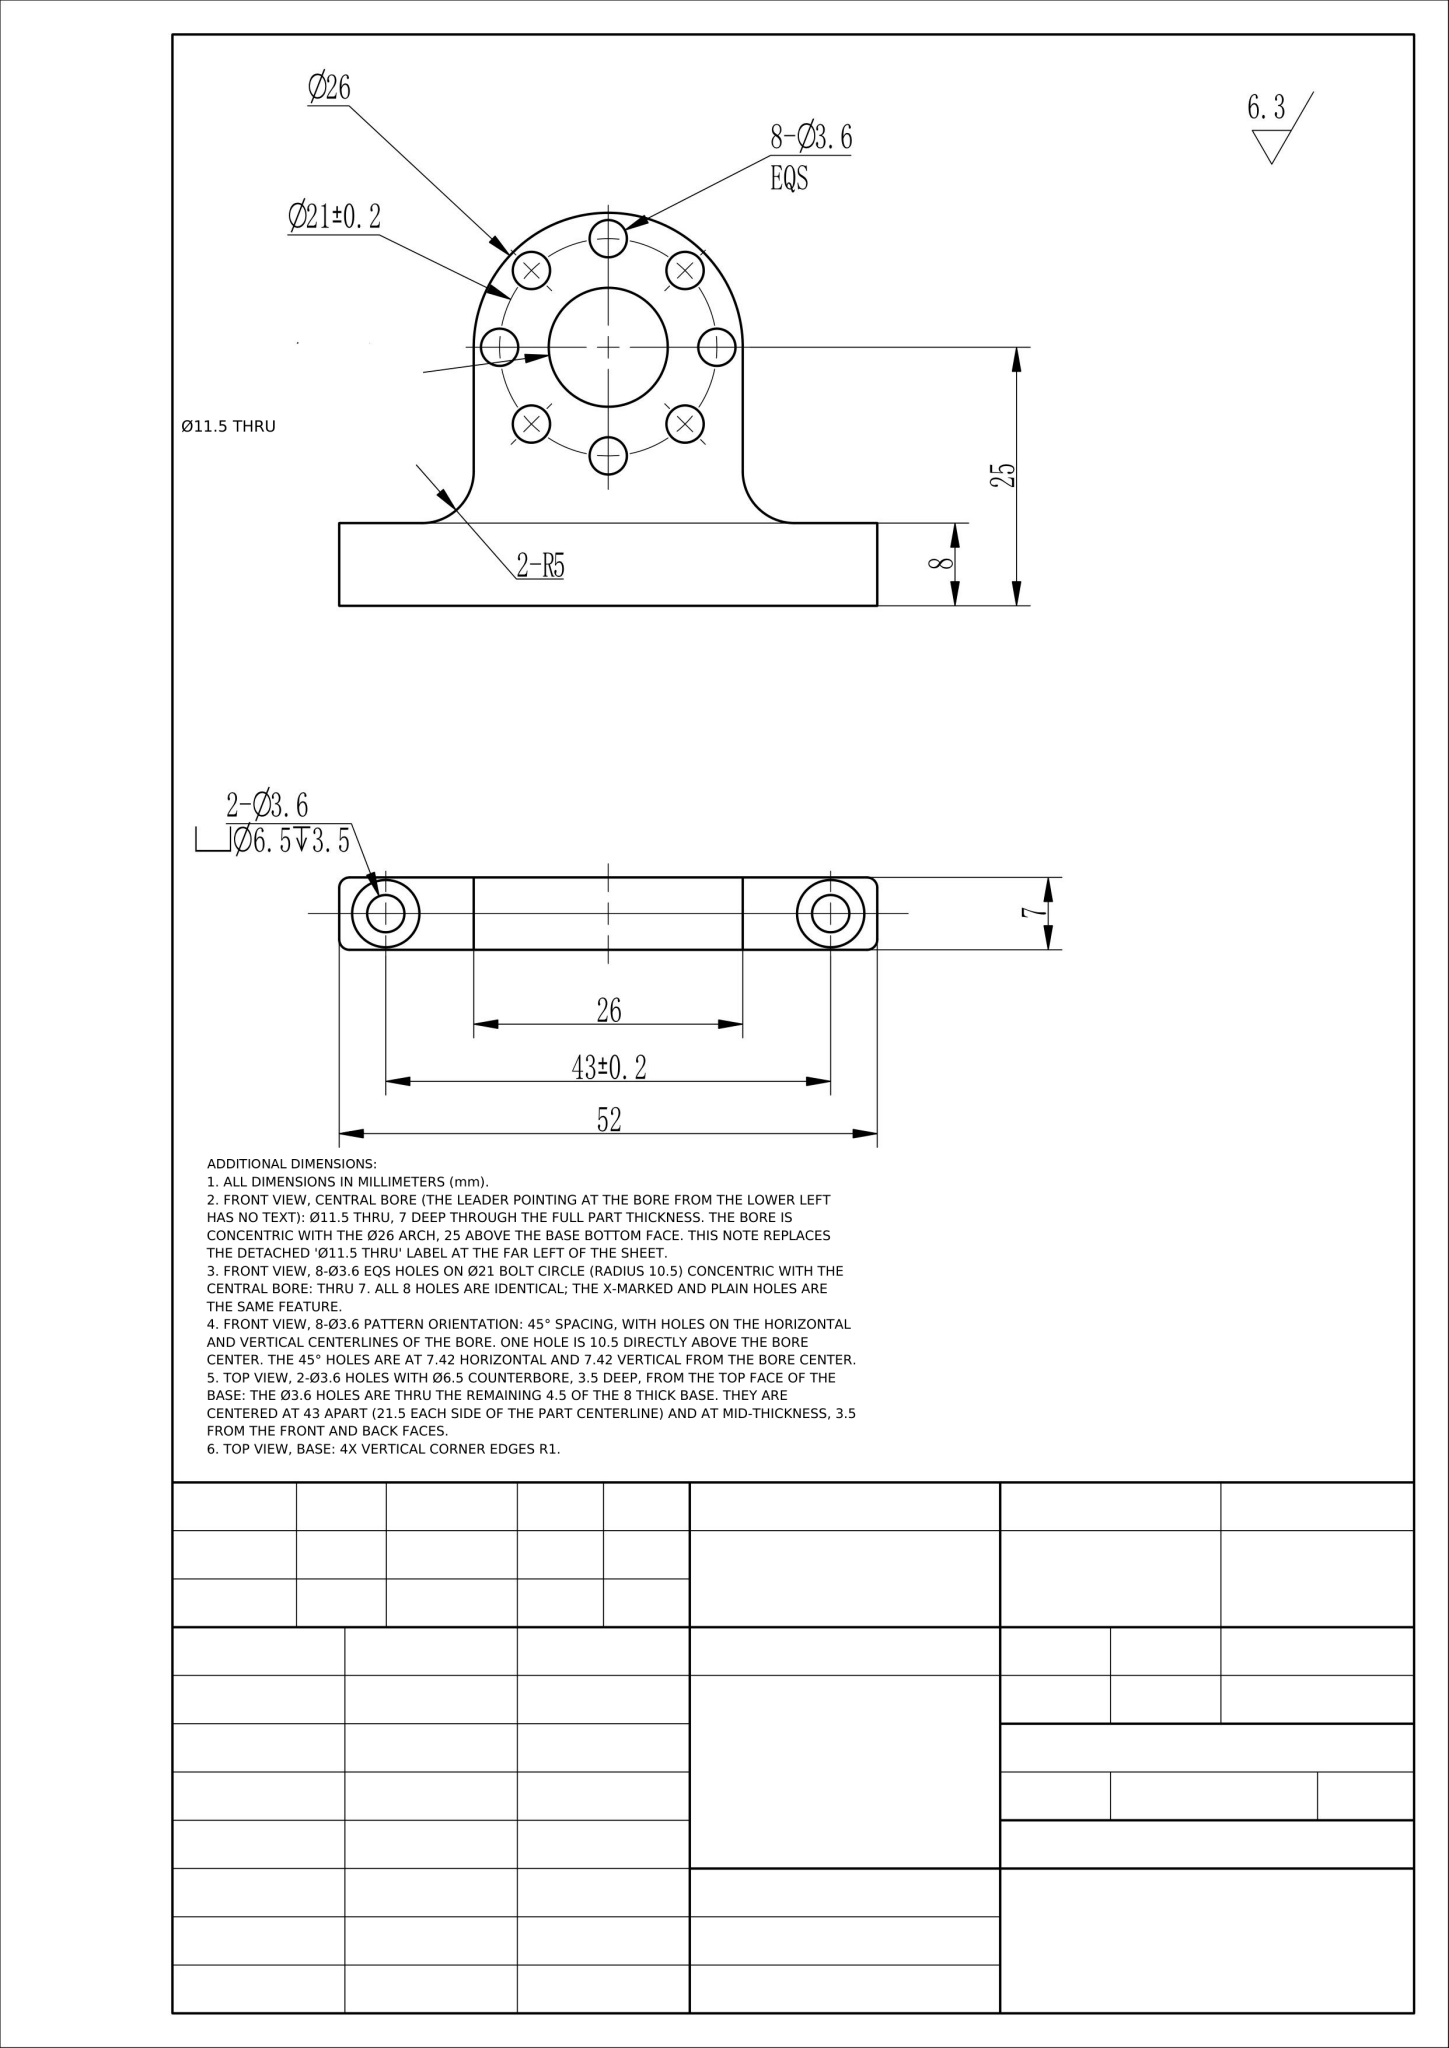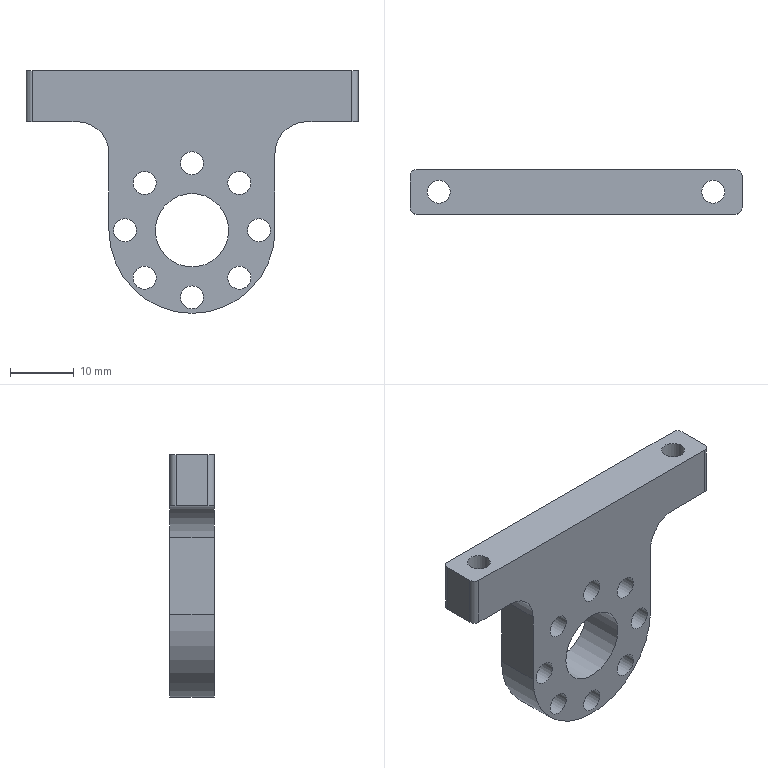Part | NX | mm | 1 solid | 31 faces | box 52 x 7 x 38 mm | volume 6312 mm3 | cylinder 20 | plane 11 | commonest cylinder face diameters 3.6 x10 2 x4 10 x2 6.5 x2 26 x1 11.5 x1
STEP:
#1=CARTESIAN_POINT('',(0.,0.,0.));
#2=DIRECTION('',(0.,0.,1.));
#3=DIRECTION('',(1.,0.,0.));
#4=AXIS2_PLACEMENT_3D('',#1,#2,#3);
#5=(LENGTH_UNIT()NAMED_UNIT(*)SI_UNIT(.MILLI.,.METRE.));
#6=UNCERTAINTY_MEASURE_WITH_UNIT(LENGTH_MEASURE(0.00002),#5,'','');
#7=(NAMED_UNIT(*)PLANE_ANGLE_UNIT()SI_UNIT($,.RADIAN.));
#8=PLANE_ANGLE_MEASURE_WITH_UNIT(PLANE_ANGLE_MEASURE(0.01745),#7);
#9=DIMENSIONAL_EXPONENTS(0.,0.,0.,0.,0.,0.,0.);
#10=(CONVERSION_BASED_UNIT('',#8)NAMED_UNIT(#9)PLANE_ANGLE_UNIT());
#11=(NAMED_UNIT(*)SI_UNIT($,.STERADIAN.)SOLID_ANGLE_UNIT());
#12=(GEOMETRIC_REPRESENTATION_CONTEXT(3)GLOBAL_UNCERTAINTY_ASSIGNED_CONTEXT((#6))GLOBAL_UNIT_ASSIGNED_CONTEXT((#5,#10,#11))REPRESENTATION_CONTEXT('',''));
#13=SHAPE_REPRESENTATION('',(#4),#12);
#14=CARTESIAN_POINT('',(-13.,-7.,-0.));
#15=VERTEX_POINT('',#14);
#16=CARTESIAN_POINT('',(13.,-7.,-0.));
#17=VERTEX_POINT('',#16);
#18=CARTESIAN_POINT('',(0.,-7.,0.));
#19=DIRECTION('',(0.,-1.,0.));
#20=DIRECTION('',(1.,0.,-0.));
#21=AXIS2_PLACEMENT_3D('',#18,#19,#20);
#22=CIRCLE('',#21,13.);
#23=EDGE_CURVE('',#15,#17,#22,.T.);
#24=ORIENTED_EDGE('',*,*,#23,.F.);
#25=CARTESIAN_POINT('',(-13.,0.,-0.));
#26=VERTEX_POINT('',#25);
#27=CARTESIAN_POINT('',(-13.,-7.,0.));
#28=DIRECTION('',(0.,1.,0.));
#29=VECTOR('',#28,1.);
#30=LINE('',#27,#29);
#31=EDGE_CURVE('',#15,#26,#30,.T.);
#32=ORIENTED_EDGE('',*,*,#31,.T.);
#33=CARTESIAN_POINT('',(13.,0.,0.));
#34=VERTEX_POINT('',#33);
#35=CARTESIAN_POINT('',(0.,0.,0.));
#36=DIRECTION('',(0.,-1.,0.));
#37=DIRECTION('',(1.,0.,-0.));
#38=AXIS2_PLACEMENT_3D('',#35,#36,#37);
#39=CIRCLE('',#38,13.);
#40=EDGE_CURVE('',#26,#34,#39,.T.);
#41=ORIENTED_EDGE('',*,*,#40,.T.);
#42=CARTESIAN_POINT('',(13.,-7.,0.));
#43=DIRECTION('',(0.,1.,0.));
#44=VECTOR('',#43,1.);
#45=LINE('',#42,#44);
#46=EDGE_CURVE('',#17,#34,#45,.T.);
#47=ORIENTED_EDGE('',*,*,#46,.F.);
#48=EDGE_LOOP('',(#24,#32,#41,#47));
#49=FACE_OUTER_BOUND('',#48,.T.);
#50=CARTESIAN_POINT('',(0.,0.,0.));
#51=DIRECTION('',(0.,-1.,0.));
#52=DIRECTION('',(0.,0.,-1.));
#53=AXIS2_PLACEMENT_3D('',#50,#51,#52);
#54=CYLINDRICAL_SURFACE('',#53,13.);
#55=ADVANCED_FACE('',(#49),#54,.T.);
#56=CARTESIAN_POINT('',(5.75,0.,-0.));
#57=VERTEX_POINT('',#56);
#58=CARTESIAN_POINT('',(0.,0.,0.));
#59=DIRECTION('',(0.,-1.,0.));
#60=DIRECTION('',(1.,0.,-0.));
#61=AXIS2_PLACEMENT_3D('',#58,#59,#60);
#62=CIRCLE('',#61,5.75);
#63=EDGE_CURVE('',#57,#57,#62,.T.);
#64=ORIENTED_EDGE('',*,*,#63,.F.);
#65=EDGE_LOOP('',(#64));
#66=FACE_BOUND('',#65,.T.);
#67=CARTESIAN_POINT('',(5.75,-7.,-0.));
#68=VERTEX_POINT('',#67);
#69=CARTESIAN_POINT('',(0.,-7.,0.));
#70=DIRECTION('',(0.,-1.,0.));
#71=DIRECTION('',(1.,0.,-0.));
#72=AXIS2_PLACEMENT_3D('',#69,#70,#71);
#73=CIRCLE('',#72,5.75);
#74=EDGE_CURVE('',#68,#68,#73,.T.);
#75=ORIENTED_EDGE('',*,*,#74,.T.);
#76=EDGE_LOOP('',(#75));
#77=FACE_BOUND('',#76,.T.);
#78=CARTESIAN_POINT('',(0.,0.,0.));
#79=DIRECTION('',(0.,-1.,0.));
#80=DIRECTION('',(0.,0.,-1.));
#81=AXIS2_PLACEMENT_3D('',#78,#79,#80);
#82=CYLINDRICAL_SURFACE('',#81,5.75);
#83=ADVANCED_FACE('',(#66,#77),#82,.F.);
#84=CARTESIAN_POINT('',(7.425,0.,5.625));
#85=VERTEX_POINT('',#84);
#86=CARTESIAN_POINT('',(7.425,0.,7.425));
#87=DIRECTION('',(0.,-1.,0.));
#88=DIRECTION('',(0.,0.,-1.));
#89=AXIS2_PLACEMENT_3D('',#86,#87,#88);
#90=CIRCLE('',#89,1.8);
#91=EDGE_CURVE('',#85,#85,#90,.T.);
#92=ORIENTED_EDGE('',*,*,#91,.T.);
#93=EDGE_LOOP('',(#92));
#94=FACE_BOUND('',#93,.T.);
#95=CARTESIAN_POINT('',(10.5,0.,-1.8));
#96=VERTEX_POINT('',#95);
#97=CARTESIAN_POINT('',(10.5,0.,-0.));
#98=DIRECTION('',(0.,-1.,0.));
#99=DIRECTION('',(0.,0.,-1.));
#100=AXIS2_PLACEMENT_3D('',#97,#98,#99);
#101=CIRCLE('',#100,1.8);
#102=EDGE_CURVE('',#96,#96,#101,.T.);
#103=ORIENTED_EDGE('',*,*,#102,.T.);
#104=EDGE_LOOP('',(#103));
#105=FACE_BOUND('',#104,.T.);
#106=CARTESIAN_POINT('',(7.425,0.,-9.225));
#107=VERTEX_POINT('',#106);
#108=CARTESIAN_POINT('',(7.425,0.,-7.425));
#109=DIRECTION('',(0.,-1.,0.));
#110=DIRECTION('',(0.,0.,-1.));
#111=AXIS2_PLACEMENT_3D('',#108,#109,#110);
#112=CIRCLE('',#111,1.8);
#113=EDGE_CURVE('',#107,#107,#112,.T.);
#114=ORIENTED_EDGE('',*,*,#113,.T.);
#115=EDGE_LOOP('',(#114));
#116=FACE_BOUND('',#115,.T.);
#117=CARTESIAN_POINT('',(0.,0.,-12.3));
#118=VERTEX_POINT('',#117);
#119=CARTESIAN_POINT('',(0.,0.,-10.5));
#120=DIRECTION('',(0.,-1.,0.));
#121=DIRECTION('',(0.,0.,-1.));
#122=AXIS2_PLACEMENT_3D('',#119,#120,#121);
#123=CIRCLE('',#122,1.8);
#124=EDGE_CURVE('',#118,#118,#123,.T.);
#125=ORIENTED_EDGE('',*,*,#124,.T.);
#126=EDGE_LOOP('',(#125));
#127=FACE_BOUND('',#126,.T.);
#128=CARTESIAN_POINT('',(-7.425,0.,-9.225));
#129=VERTEX_POINT('',#128);
#130=CARTESIAN_POINT('',(-7.425,0.,-7.425));
#131=DIRECTION('',(0.,-1.,0.));
#132=DIRECTION('',(0.,0.,-1.));
#133=AXIS2_PLACEMENT_3D('',#130,#131,#132);
#134=CIRCLE('',#133,1.8);
#135=EDGE_CURVE('',#129,#129,#134,.T.);
#136=ORIENTED_EDGE('',*,*,#135,.T.);
#137=EDGE_LOOP('',(#136));
#138=FACE_BOUND('',#137,.T.);
#139=CARTESIAN_POINT('',(-10.5,0.,-1.8));
#140=VERTEX_POINT('',#139);
#141=CARTESIAN_POINT('',(-10.5,0.,0.));
#142=DIRECTION('',(0.,-1.,0.));
#143=DIRECTION('',(0.,0.,-1.));
#144=AXIS2_PLACEMENT_3D('',#141,#142,#143);
#145=CIRCLE('',#144,1.8);
#146=EDGE_CURVE('',#140,#140,#145,.T.);
#147=ORIENTED_EDGE('',*,*,#146,.T.);
#148=EDGE_LOOP('',(#147));
#149=FACE_BOUND('',#148,.T.);
#150=CARTESIAN_POINT('',(-7.425,0.,5.625));
#151=VERTEX_POINT('',#150);
#152=CARTESIAN_POINT('',(-7.425,0.,7.425));
#153=DIRECTION('',(0.,-1.,0.));
#154=DIRECTION('',(0.,0.,-1.));
#155=AXIS2_PLACEMENT_3D('',#152,#153,#154);
#156=CIRCLE('',#155,1.8);
#157=EDGE_CURVE('',#151,#151,#156,.T.);
#158=ORIENTED_EDGE('',*,*,#157,.T.);
#159=EDGE_LOOP('',(#158));
#160=FACE_BOUND('',#159,.T.);
#161=CARTESIAN_POINT('',(0.,0.,8.7));
#162=VERTEX_POINT('',#161);
#163=CARTESIAN_POINT('',(0.,0.,10.5));
#164=DIRECTION('',(0.,-1.,0.));
#165=DIRECTION('',(0.,0.,-1.));
#166=AXIS2_PLACEMENT_3D('',#163,#164,#165);
#167=CIRCLE('',#166,1.8);
#168=EDGE_CURVE('',#162,#162,#167,.T.);
#169=ORIENTED_EDGE('',*,*,#168,.T.);
#170=EDGE_LOOP('',(#169));
#171=FACE_BOUND('',#170,.T.);
#172=CARTESIAN_POINT('',(25.,0.,25.));
#173=VERTEX_POINT('',#172);
#174=CARTESIAN_POINT('',(-25.,0.,25.));
#175=VERTEX_POINT('',#174);
#176=CARTESIAN_POINT('',(26.,0.,25.));
#177=DIRECTION('',(-1.,0.,0.));
#178=VECTOR('',#177,1.);
#179=LINE('',#176,#178);
#180=EDGE_CURVE('',#173,#175,#179,.T.);
#181=ORIENTED_EDGE('',*,*,#180,.F.);
#182=CARTESIAN_POINT('',(25.,0.,17.));
#183=VERTEX_POINT('',#182);
#184=CARTESIAN_POINT('',(25.,0.,0.));
#185=DIRECTION('',(0.,0.,-1.));
#186=VECTOR('',#185,1.);
#187=LINE('',#184,#186);
#188=EDGE_CURVE('',#173,#183,#187,.T.);
#189=ORIENTED_EDGE('',*,*,#188,.T.);
#190=CARTESIAN_POINT('',(18.,0.,17.));
#191=VERTEX_POINT('',#190);
#192=CARTESIAN_POINT('',(13.,0.,17.));
#193=DIRECTION('',(1.,0.,0.));
#194=VECTOR('',#193,1.);
#195=LINE('',#192,#194);
#196=EDGE_CURVE('',#191,#183,#195,.T.);
#197=ORIENTED_EDGE('',*,*,#196,.F.);
#198=CARTESIAN_POINT('',(13.,0.,12.));
#199=VERTEX_POINT('',#198);
#200=CARTESIAN_POINT('',(18.,0.,12.));
#201=DIRECTION('',(0.,-1.,0.));
#202=DIRECTION('',(0.,0.,-1.));
#203=AXIS2_PLACEMENT_3D('',#200,#201,#202);
#204=CIRCLE('',#203,5.);
#205=EDGE_CURVE('',#191,#199,#204,.T.);
#206=ORIENTED_EDGE('',*,*,#205,.T.);
#207=CARTESIAN_POINT('',(13.,0.,0.));
#208=DIRECTION('',(0.,0.,1.));
#209=VECTOR('',#208,1.);
#210=LINE('',#207,#209);
#211=EDGE_CURVE('',#34,#199,#210,.T.);
#212=ORIENTED_EDGE('',*,*,#211,.F.);
#213=ORIENTED_EDGE('',*,*,#40,.F.);
#214=CARTESIAN_POINT('',(-13.,0.,12.));
#215=VERTEX_POINT('',#214);
#216=CARTESIAN_POINT('',(-13.,0.,17.));
#217=DIRECTION('',(0.,0.,-1.));
#218=VECTOR('',#217,1.);
#219=LINE('',#216,#218);
#220=EDGE_CURVE('',#215,#26,#219,.T.);
#221=ORIENTED_EDGE('',*,*,#220,.F.);
#222=CARTESIAN_POINT('',(-18.,0.,17.));
#223=VERTEX_POINT('',#222);
#224=CARTESIAN_POINT('',(-18.,0.,12.));
#225=DIRECTION('',(0.,-1.,0.));
#226=DIRECTION('',(0.,0.,-1.));
#227=AXIS2_PLACEMENT_3D('',#224,#225,#226);
#228=CIRCLE('',#227,5.);
#229=EDGE_CURVE('',#215,#223,#228,.T.);
#230=ORIENTED_EDGE('',*,*,#229,.T.);
#231=CARTESIAN_POINT('',(-25.,0.,17.));
#232=VERTEX_POINT('',#231);
#233=CARTESIAN_POINT('',(-26.,0.,17.));
#234=DIRECTION('',(1.,0.,0.));
#235=VECTOR('',#234,1.);
#236=LINE('',#233,#235);
#237=EDGE_CURVE('',#232,#223,#236,.T.);
#238=ORIENTED_EDGE('',*,*,#237,.F.);
#239=CARTESIAN_POINT('',(-25.,0.,0.));
#240=DIRECTION('',(0.,0.,1.));
#241=VECTOR('',#240,1.);
#242=LINE('',#239,#241);
#243=EDGE_CURVE('',#232,#175,#242,.T.);
#244=ORIENTED_EDGE('',*,*,#243,.T.);
#245=EDGE_LOOP('',(#181,#189,#197,#206,#212,#213,#221,#230,#238,#244));
#246=FACE_BOUND('',#245,.T.);
#247=ORIENTED_EDGE('',*,*,#63,.T.);
#248=EDGE_LOOP('',(#247));
#249=FACE_BOUND('',#248,.T.);
#250=CARTESIAN_POINT('',(0.,0.,0.));
#251=DIRECTION('',(0.,-1.,0.));
#252=DIRECTION('',(0.,0.,-1.));
#253=AXIS2_PLACEMENT_3D('',#250,#251,#252);
#254=PLANE('',#253);
#255=ADVANCED_FACE('',(#94,#105,#116,#127,#138,#149,#160,#171,#246,#249),#254,.F.);
#256=CARTESIAN_POINT('',(7.425,-7.,9.225));
#257=VERTEX_POINT('',#256);
#258=CARTESIAN_POINT('',(7.425,-7.,7.425));
#259=DIRECTION('',(0.,1.,0.));
#260=DIRECTION('',(0.,0.,1.));
#261=AXIS2_PLACEMENT_3D('',#258,#259,#260);
#262=CIRCLE('',#261,1.8);
#263=EDGE_CURVE('',#257,#257,#262,.T.);
#264=ORIENTED_EDGE('',*,*,#263,.T.);
#265=EDGE_LOOP('',(#264));
#266=FACE_BOUND('',#265,.T.);
#267=CARTESIAN_POINT('',(10.5,-7.,1.8));
#268=VERTEX_POINT('',#267);
#269=CARTESIAN_POINT('',(10.5,-7.,-0.));
#270=DIRECTION('',(0.,1.,0.));
#271=DIRECTION('',(0.,0.,1.));
#272=AXIS2_PLACEMENT_3D('',#269,#270,#271);
#273=CIRCLE('',#272,1.8);
#274=EDGE_CURVE('',#268,#268,#273,.T.);
#275=ORIENTED_EDGE('',*,*,#274,.T.);
#276=EDGE_LOOP('',(#275));
#277=FACE_BOUND('',#276,.T.);
#278=CARTESIAN_POINT('',(7.425,-7.,-5.625));
#279=VERTEX_POINT('',#278);
#280=CARTESIAN_POINT('',(7.425,-7.,-7.425));
#281=DIRECTION('',(0.,1.,0.));
#282=DIRECTION('',(0.,0.,1.));
#283=AXIS2_PLACEMENT_3D('',#280,#281,#282);
#284=CIRCLE('',#283,1.8);
#285=EDGE_CURVE('',#279,#279,#284,.T.);
#286=ORIENTED_EDGE('',*,*,#285,.T.);
#287=EDGE_LOOP('',(#286));
#288=FACE_BOUND('',#287,.T.);
#289=CARTESIAN_POINT('',(0.,-7.,-8.7));
#290=VERTEX_POINT('',#289);
#291=CARTESIAN_POINT('',(0.,-7.,-10.5));
#292=DIRECTION('',(0.,1.,0.));
#293=DIRECTION('',(0.,0.,1.));
#294=AXIS2_PLACEMENT_3D('',#291,#292,#293);
#295=CIRCLE('',#294,1.8);
#296=EDGE_CURVE('',#290,#290,#295,.T.);
#297=ORIENTED_EDGE('',*,*,#296,.T.);
#298=EDGE_LOOP('',(#297));
#299=FACE_BOUND('',#298,.T.);
#300=CARTESIAN_POINT('',(-7.425,-7.,-5.625));
#301=VERTEX_POINT('',#300);
#302=CARTESIAN_POINT('',(-7.425,-7.,-7.425));
#303=DIRECTION('',(0.,1.,0.));
#304=DIRECTION('',(0.,0.,1.));
#305=AXIS2_PLACEMENT_3D('',#302,#303,#304);
#306=CIRCLE('',#305,1.8);
#307=EDGE_CURVE('',#301,#301,#306,.T.);
#308=ORIENTED_EDGE('',*,*,#307,.T.);
#309=EDGE_LOOP('',(#308));
#310=FACE_BOUND('',#309,.T.);
#311=CARTESIAN_POINT('',(-10.5,-7.,1.8));
#312=VERTEX_POINT('',#311);
#313=CARTESIAN_POINT('',(-10.5,-7.,0.));
#314=DIRECTION('',(0.,1.,0.));
#315=DIRECTION('',(0.,0.,1.));
#316=AXIS2_PLACEMENT_3D('',#313,#314,#315);
#317=CIRCLE('',#316,1.8);
#318=EDGE_CURVE('',#312,#312,#317,.T.);
#319=ORIENTED_EDGE('',*,*,#318,.T.);
#320=EDGE_LOOP('',(#319));
#321=FACE_BOUND('',#320,.T.);
#322=CARTESIAN_POINT('',(-7.425,-7.,9.225));
#323=VERTEX_POINT('',#322);
#324=CARTESIAN_POINT('',(-7.425,-7.,7.425));
#325=DIRECTION('',(0.,1.,0.));
#326=DIRECTION('',(0.,0.,1.));
#327=AXIS2_PLACEMENT_3D('',#324,#325,#326);
#328=CIRCLE('',#327,1.8);
#329=EDGE_CURVE('',#323,#323,#328,.T.);
#330=ORIENTED_EDGE('',*,*,#329,.T.);
#331=EDGE_LOOP('',(#330));
#332=FACE_BOUND('',#331,.T.);
#333=CARTESIAN_POINT('',(0.,-7.,12.3));
#334=VERTEX_POINT('',#333);
#335=CARTESIAN_POINT('',(0.,-7.,10.5));
#336=DIRECTION('',(0.,1.,0.));
#337=DIRECTION('',(0.,0.,1.));
#338=AXIS2_PLACEMENT_3D('',#335,#336,#337);
#339=CIRCLE('',#338,1.8);
#340=EDGE_CURVE('',#334,#334,#339,.T.);
#341=ORIENTED_EDGE('',*,*,#340,.T.);
#342=EDGE_LOOP('',(#341));
#343=FACE_BOUND('',#342,.T.);
#344=ORIENTED_EDGE('',*,*,#74,.F.);
#345=EDGE_LOOP('',(#344));
#346=FACE_BOUND('',#345,.T.);
#347=CARTESIAN_POINT('',(18.,-7.,17.));
#348=VERTEX_POINT('',#347);
#349=CARTESIAN_POINT('',(25.,-7.,17.));
#350=VERTEX_POINT('',#349);
#351=CARTESIAN_POINT('',(13.,-7.,17.));
#352=DIRECTION('',(1.,0.,0.));
#353=VECTOR('',#352,1.);
#354=LINE('',#351,#353);
#355=EDGE_CURVE('',#348,#350,#354,.T.);
#356=ORIENTED_EDGE('',*,*,#355,.T.);
#357=CARTESIAN_POINT('',(25.,-7.,25.));
#358=VERTEX_POINT('',#357);
#359=CARTESIAN_POINT('',(25.,-7.,25.));
#360=DIRECTION('',(0.,0.,1.));
#361=VECTOR('',#360,1.);
#362=LINE('',#359,#361);
#363=EDGE_CURVE('',#350,#358,#362,.T.);
#364=ORIENTED_EDGE('',*,*,#363,.T.);
#365=CARTESIAN_POINT('',(-25.,-7.,25.));
#366=VERTEX_POINT('',#365);
#367=CARTESIAN_POINT('',(26.,-7.,25.));
#368=DIRECTION('',(-1.,0.,0.));
#369=VECTOR('',#368,1.);
#370=LINE('',#367,#369);
#371=EDGE_CURVE('',#358,#366,#370,.T.);
#372=ORIENTED_EDGE('',*,*,#371,.T.);
#373=CARTESIAN_POINT('',(-25.,-7.,17.));
#374=VERTEX_POINT('',#373);
#375=CARTESIAN_POINT('',(-25.,-7.,17.));
#376=DIRECTION('',(0.,0.,-1.));
#377=VECTOR('',#376,1.);
#378=LINE('',#375,#377);
#379=EDGE_CURVE('',#366,#374,#378,.T.);
#380=ORIENTED_EDGE('',*,*,#379,.T.);
#381=CARTESIAN_POINT('',(-18.,-7.,17.));
#382=VERTEX_POINT('',#381);
#383=CARTESIAN_POINT('',(-26.,-7.,17.));
#384=DIRECTION('',(1.,0.,0.));
#385=VECTOR('',#384,1.);
#386=LINE('',#383,#385);
#387=EDGE_CURVE('',#374,#382,#386,.T.);
#388=ORIENTED_EDGE('',*,*,#387,.T.);
#389=CARTESIAN_POINT('',(-13.,-7.,12.));
#390=VERTEX_POINT('',#389);
#391=CARTESIAN_POINT('',(-18.,-7.,12.));
#392=DIRECTION('',(0.,1.,0.));
#393=DIRECTION('',(0.,0.,-1.));
#394=AXIS2_PLACEMENT_3D('',#391,#392,#393);
#395=CIRCLE('',#394,5.);
#396=EDGE_CURVE('',#382,#390,#395,.T.);
#397=ORIENTED_EDGE('',*,*,#396,.T.);
#398=CARTESIAN_POINT('',(-13.,-7.,17.));
#399=DIRECTION('',(0.,0.,-1.));
#400=VECTOR('',#399,1.);
#401=LINE('',#398,#400);
#402=EDGE_CURVE('',#390,#15,#401,.T.);
#403=ORIENTED_EDGE('',*,*,#402,.T.);
#404=ORIENTED_EDGE('',*,*,#23,.T.);
#405=CARTESIAN_POINT('',(13.,-7.,12.));
#406=VERTEX_POINT('',#405);
#407=CARTESIAN_POINT('',(13.,-7.,0.));
#408=DIRECTION('',(0.,0.,1.));
#409=VECTOR('',#408,1.);
#410=LINE('',#407,#409);
#411=EDGE_CURVE('',#17,#406,#410,.T.);
#412=ORIENTED_EDGE('',*,*,#411,.T.);
#413=CARTESIAN_POINT('',(18.,-7.,12.));
#414=DIRECTION('',(0.,1.,0.));
#415=DIRECTION('',(0.,0.,-1.));
#416=AXIS2_PLACEMENT_3D('',#413,#414,#415);
#417=CIRCLE('',#416,5.);
#418=EDGE_CURVE('',#406,#348,#417,.T.);
#419=ORIENTED_EDGE('',*,*,#418,.T.);
#420=EDGE_LOOP('',(#356,#364,#372,#380,#388,#397,#403,#404,#412,#419));
#421=FACE_BOUND('',#420,.T.);
#422=CARTESIAN_POINT('',(0.,-7.,0.));
#423=DIRECTION('',(0.,-1.,0.));
#424=DIRECTION('',(0.,0.,-1.));
#425=AXIS2_PLACEMENT_3D('',#422,#423,#424);
#426=PLANE('',#425);
#427=ADVANCED_FACE('',(#266,#277,#288,#299,#310,#321,#332,#343,#346,#421),#426,.T.);
#428=CARTESIAN_POINT('',(-26.,-6.,25.));
#429=VERTEX_POINT('',#428);
#430=CARTESIAN_POINT('',(-26.,-1.,25.));
#431=VERTEX_POINT('',#430);
#432=CARTESIAN_POINT('',(-26.,-7.,25.));
#433=DIRECTION('',(0.,1.,0.));
#434=VECTOR('',#433,1.);
#435=LINE('',#432,#434);
#436=EDGE_CURVE('',#429,#431,#435,.T.);
#437=ORIENTED_EDGE('',*,*,#436,.T.);
#438=CARTESIAN_POINT('',(-26.,-1.,17.));
#439=VERTEX_POINT('',#438);
#440=CARTESIAN_POINT('',(-26.,-1.,25.));
#441=DIRECTION('',(0.,0.,-1.));
#442=VECTOR('',#441,1.);
#443=LINE('',#440,#442);
#444=EDGE_CURVE('',#431,#439,#443,.T.);
#445=ORIENTED_EDGE('',*,*,#444,.T.);
#446=CARTESIAN_POINT('',(-26.,-6.,17.));
#447=VERTEX_POINT('',#446);
#448=CARTESIAN_POINT('',(-26.,-7.,17.));
#449=DIRECTION('',(0.,1.,0.));
#450=VECTOR('',#449,1.);
#451=LINE('',#448,#450);
#452=EDGE_CURVE('',#447,#439,#451,.T.);
#453=ORIENTED_EDGE('',*,*,#452,.F.);
#454=CARTESIAN_POINT('',(-26.,-6.,25.));
#455=DIRECTION('',(0.,0.,1.));
#456=VECTOR('',#455,1.);
#457=LINE('',#454,#456);
#458=EDGE_CURVE('',#447,#429,#457,.T.);
#459=ORIENTED_EDGE('',*,*,#458,.T.);
#460=EDGE_LOOP('',(#437,#445,#453,#459));
#461=FACE_OUTER_BOUND('',#460,.T.);
#462=CARTESIAN_POINT('',(-26.,-7.,25.));
#463=DIRECTION('',(1.,0.,0.));
#464=DIRECTION('',(0.,0.,-1.));
#465=AXIS2_PLACEMENT_3D('',#462,#463,#464);
#466=PLANE('',#465);
#467=ADVANCED_FACE('',(#461),#466,.F.);
#468=CARTESIAN_POINT('',(-18.25,-3.5,17.));
#469=VERTEX_POINT('',#468);
#470=CARTESIAN_POINT('',(-21.5,-3.5,17.));
#471=DIRECTION('',(0.,0.,1.));
#472=DIRECTION('',(1.,0.,0.));
#473=AXIS2_PLACEMENT_3D('',#470,#471,#472);
#474=CIRCLE('',#473,3.25);
#475=EDGE_CURVE('',#469,#469,#474,.T.);
#476=ORIENTED_EDGE('',*,*,#475,.T.);
#477=EDGE_LOOP('',(#476));
#478=FACE_BOUND('',#477,.T.);
#479=ORIENTED_EDGE('',*,*,#452,.T.);
#480=CARTESIAN_POINT('',(-25.,-1.,17.));
#481=DIRECTION('',(0.,0.,-1.));
#482=DIRECTION('',(1.,0.,0.));
#483=AXIS2_PLACEMENT_3D('',#480,#481,#482);
#484=CIRCLE('',#483,1.);
#485=EDGE_CURVE('',#439,#232,#484,.T.);
#486=ORIENTED_EDGE('',*,*,#485,.T.);
#487=ORIENTED_EDGE('',*,*,#237,.T.);
#488=CARTESIAN_POINT('',(-18.,-7.,17.));
#489=DIRECTION('',(0.,-1.,0.));
#490=VECTOR('',#489,1.);
#491=LINE('',#488,#490);
#492=EDGE_CURVE('',#223,#382,#491,.T.);
#493=ORIENTED_EDGE('',*,*,#492,.T.);
#494=ORIENTED_EDGE('',*,*,#387,.F.);
#495=CARTESIAN_POINT('',(-25.,-6.,17.));
#496=DIRECTION('',(0.,0.,-1.));
#497=DIRECTION('',(1.,0.,0.));
#498=AXIS2_PLACEMENT_3D('',#495,#496,#497);
#499=CIRCLE('',#498,1.);
#500=EDGE_CURVE('',#374,#447,#499,.T.);
#501=ORIENTED_EDGE('',*,*,#500,.T.);
#502=EDGE_LOOP('',(#479,#486,#487,#493,#494,#501));
#503=FACE_BOUND('',#502,.T.);
#504=CARTESIAN_POINT('',(-26.,-7.,17.));
#505=DIRECTION('',(0.,0.,1.));
#506=DIRECTION('',(1.,0.,0.));
#507=AXIS2_PLACEMENT_3D('',#504,#505,#506);
#508=PLANE('',#507);
#509=ADVANCED_FACE('',(#478,#503),#508,.F.);
#510=ORIENTED_EDGE('',*,*,#402,.F.);
#511=CARTESIAN_POINT('',(-13.,0.,12.));
#512=DIRECTION('',(0.,1.,0.));
#513=VECTOR('',#512,1.);
#514=LINE('',#511,#513);
#515=EDGE_CURVE('',#390,#215,#514,.T.);
#516=ORIENTED_EDGE('',*,*,#515,.T.);
#517=ORIENTED_EDGE('',*,*,#220,.T.);
#518=ORIENTED_EDGE('',*,*,#31,.F.);
#519=EDGE_LOOP('',(#510,#516,#517,#518));
#520=FACE_OUTER_BOUND('',#519,.T.);
#521=CARTESIAN_POINT('',(-13.,-7.,17.));
#522=DIRECTION('',(1.,0.,0.));
#523=DIRECTION('',(0.,0.,-1.));
#524=AXIS2_PLACEMENT_3D('',#521,#522,#523);
#525=PLANE('',#524);
#526=ADVANCED_FACE('',(#520),#525,.F.);
#527=ORIENTED_EDGE('',*,*,#211,.T.);
#528=CARTESIAN_POINT('',(13.,-7.,12.));
#529=DIRECTION('',(0.,-1.,0.));
#530=VECTOR('',#529,1.);
#531=LINE('',#528,#530);
#532=EDGE_CURVE('',#199,#406,#531,.T.);
#533=ORIENTED_EDGE('',*,*,#532,.T.);
#534=ORIENTED_EDGE('',*,*,#411,.F.);
#535=ORIENTED_EDGE('',*,*,#46,.T.);
#536=EDGE_LOOP('',(#527,#533,#534,#535));
#537=FACE_OUTER_BOUND('',#536,.T.);
#538=CARTESIAN_POINT('',(13.,-7.,0.));
#539=DIRECTION('',(-1.,0.,0.));
#540=DIRECTION('',(0.,0.,1.));
#541=AXIS2_PLACEMENT_3D('',#538,#539,#540);
#542=PLANE('',#541);
#543=ADVANCED_FACE('',(#537),#542,.F.);
#544=CARTESIAN_POINT('',(24.75,-3.5,17.));
#545=VERTEX_POINT('',#544);
#546=CARTESIAN_POINT('',(21.5,-3.5,17.));
#547=DIRECTION('',(0.,0.,1.));
#548=DIRECTION('',(1.,0.,0.));
#549=AXIS2_PLACEMENT_3D('',#546,#547,#548);
#550=CIRCLE('',#549,3.25);
#551=EDGE_CURVE('',#545,#545,#550,.T.);
#552=ORIENTED_EDGE('',*,*,#551,.T.);
#553=EDGE_LOOP('',(#552));
#554=FACE_BOUND('',#553,.T.);
#555=ORIENTED_EDGE('',*,*,#196,.T.);
#556=CARTESIAN_POINT('',(26.,-1.,17.));
#557=VERTEX_POINT('',#556);
#558=CARTESIAN_POINT('',(25.,-1.,17.));
#559=DIRECTION('',(0.,0.,-1.));
#560=DIRECTION('',(1.,0.,0.));
#561=AXIS2_PLACEMENT_3D('',#558,#559,#560);
#562=CIRCLE('',#561,1.);
#563=EDGE_CURVE('',#183,#557,#562,.T.);
#564=ORIENTED_EDGE('',*,*,#563,.T.);
#565=CARTESIAN_POINT('',(26.,-6.,17.));
#566=VERTEX_POINT('',#565);
#567=CARTESIAN_POINT('',(26.,-7.,17.));
#568=DIRECTION('',(0.,1.,0.));
#569=VECTOR('',#568,1.);
#570=LINE('',#567,#569);
#571=EDGE_CURVE('',#566,#557,#570,.T.);
#572=ORIENTED_EDGE('',*,*,#571,.F.);
#573=CARTESIAN_POINT('',(25.,-6.,17.));
#574=DIRECTION('',(0.,0.,-1.));
#575=DIRECTION('',(1.,0.,0.));
#576=AXIS2_PLACEMENT_3D('',#573,#574,#575);
#577=CIRCLE('',#576,1.);
#578=EDGE_CURVE('',#566,#350,#577,.T.);
#579=ORIENTED_EDGE('',*,*,#578,.T.);
#580=ORIENTED_EDGE('',*,*,#355,.F.);
#581=CARTESIAN_POINT('',(18.,0.,17.));
#582=DIRECTION('',(0.,1.,0.));
#583=VECTOR('',#582,1.);
#584=LINE('',#581,#583);
#585=EDGE_CURVE('',#348,#191,#584,.T.);
#586=ORIENTED_EDGE('',*,*,#585,.T.);
#587=EDGE_LOOP('',(#555,#564,#572,#579,#580,#586));
#588=FACE_BOUND('',#587,.T.);
#589=CARTESIAN_POINT('',(13.,-7.,17.));
#590=DIRECTION('',(0.,0.,1.));
#591=DIRECTION('',(1.,0.,0.));
#592=AXIS2_PLACEMENT_3D('',#589,#590,#591);
#593=PLANE('',#592);
#594=ADVANCED_FACE('',(#554,#588),#593,.F.);
#595=ORIENTED_EDGE('',*,*,#571,.T.);
#596=CARTESIAN_POINT('',(26.,-1.,25.));
#597=VERTEX_POINT('',#596);
#598=CARTESIAN_POINT('',(26.,-1.,17.));
#599=DIRECTION('',(0.,0.,1.));
#600=VECTOR('',#599,1.);
#601=LINE('',#598,#600);
#602=EDGE_CURVE('',#557,#597,#601,.T.);
#603=ORIENTED_EDGE('',*,*,#602,.T.);
#604=CARTESIAN_POINT('',(26.,-6.,25.));
#605=VERTEX_POINT('',#604);
#606=CARTESIAN_POINT('',(26.,-7.,25.));
#607=DIRECTION('',(0.,1.,0.));
#608=VECTOR('',#607,1.);
#609=LINE('',#606,#608);
#610=EDGE_CURVE('',#605,#597,#609,.T.);
#611=ORIENTED_EDGE('',*,*,#610,.F.);
#612=CARTESIAN_POINT('',(26.,-6.,17.));
#613=DIRECTION('',(0.,0.,-1.));
#614=VECTOR('',#613,1.);
#615=LINE('',#612,#614);
#616=EDGE_CURVE('',#605,#566,#615,.T.);
#617=ORIENTED_EDGE('',*,*,#616,.T.);
#618=EDGE_LOOP('',(#595,#603,#611,#617));
#619=FACE_OUTER_BOUND('',#618,.T.);
#620=CARTESIAN_POINT('',(26.,-7.,17.));
#621=DIRECTION('',(-1.,0.,0.));
#622=DIRECTION('',(0.,0.,1.));
#623=AXIS2_PLACEMENT_3D('',#620,#621,#622);
#624=PLANE('',#623);
#625=ADVANCED_FACE('',(#619),#624,.F.);
#626=CARTESIAN_POINT('',(19.7,-3.5,25.));
#627=VERTEX_POINT('',#626);
#628=CARTESIAN_POINT('',(21.5,-3.5,25.));
#629=DIRECTION('',(0.,0.,-1.));
#630=DIRECTION('',(-1.,0.,0.));
#631=AXIS2_PLACEMENT_3D('',#628,#629,#630);
#632=CIRCLE('',#631,1.8);
#633=EDGE_CURVE('',#627,#627,#632,.T.);
#634=ORIENTED_EDGE('',*,*,#633,.T.);
#635=EDGE_LOOP('',(#634));
#636=FACE_BOUND('',#635,.T.);
#637=CARTESIAN_POINT('',(-23.3,-3.5,25.));
#638=VERTEX_POINT('',#637);
#639=CARTESIAN_POINT('',(-21.5,-3.5,25.));
#640=DIRECTION('',(0.,0.,-1.));
#641=DIRECTION('',(-1.,0.,0.));
#642=AXIS2_PLACEMENT_3D('',#639,#640,#641);
#643=CIRCLE('',#642,1.8);
#644=EDGE_CURVE('',#638,#638,#643,.T.);
#645=ORIENTED_EDGE('',*,*,#644,.T.);
#646=EDGE_LOOP('',(#645));
#647=FACE_BOUND('',#646,.T.);
#648=ORIENTED_EDGE('',*,*,#610,.T.);
#649=CARTESIAN_POINT('',(25.,-1.,25.));
#650=DIRECTION('',(0.,0.,1.));
#651=DIRECTION('',(-1.,0.,0.));
#652=AXIS2_PLACEMENT_3D('',#649,#650,#651);
#653=CIRCLE('',#652,1.);
#654=EDGE_CURVE('',#597,#173,#653,.T.);
#655=ORIENTED_EDGE('',*,*,#654,.T.);
#656=ORIENTED_EDGE('',*,*,#180,.T.);
#657=CARTESIAN_POINT('',(-25.,-1.,25.));
#658=DIRECTION('',(0.,0.,1.));
#659=DIRECTION('',(-1.,0.,0.));
#660=AXIS2_PLACEMENT_3D('',#657,#658,#659);
#661=CIRCLE('',#660,1.);
#662=EDGE_CURVE('',#175,#431,#661,.T.);
#663=ORIENTED_EDGE('',*,*,#662,.T.);
#664=ORIENTED_EDGE('',*,*,#436,.F.);
#665=CARTESIAN_POINT('',(-25.,-6.,25.));
#666=DIRECTION('',(0.,0.,1.));
#667=DIRECTION('',(-1.,0.,0.));
#668=AXIS2_PLACEMENT_3D('',#665,#666,#667);
#669=CIRCLE('',#668,1.);
#670=EDGE_CURVE('',#429,#366,#669,.T.);
#671=ORIENTED_EDGE('',*,*,#670,.T.);
#672=ORIENTED_EDGE('',*,*,#371,.F.);
#673=CARTESIAN_POINT('',(25.,-6.,25.));
#674=DIRECTION('',(0.,0.,1.));
#675=DIRECTION('',(-1.,0.,0.));
#676=AXIS2_PLACEMENT_3D('',#673,#674,#675);
#677=CIRCLE('',#676,1.);
#678=EDGE_CURVE('',#358,#605,#677,.T.);
#679=ORIENTED_EDGE('',*,*,#678,.T.);
#680=EDGE_LOOP('',(#648,#655,#656,#663,#664,#671,#672,#679));
#681=FACE_BOUND('',#680,.T.);
#682=CARTESIAN_POINT('',(26.,-7.,25.));
#683=DIRECTION('',(0.,0.,-1.));
#684=DIRECTION('',(-1.,0.,0.));
#685=AXIS2_PLACEMENT_3D('',#682,#683,#684);
#686=PLANE('',#685);
#687=ADVANCED_FACE('',(#636,#647,#681),#686,.F.);
#688=ORIENTED_EDGE('',*,*,#340,.F.);
#689=EDGE_LOOP('',(#688));
#690=FACE_BOUND('',#689,.T.);
#691=ORIENTED_EDGE('',*,*,#168,.F.);
#692=EDGE_LOOP('',(#691));
#693=FACE_BOUND('',#692,.T.);
#694=CARTESIAN_POINT('',(0.,-7.,10.5));
#695=DIRECTION('',(0.,1.,0.));
#696=DIRECTION('',(0.,0.,1.));
#697=AXIS2_PLACEMENT_3D('',#694,#695,#696);
#698=CYLINDRICAL_SURFACE('',#697,1.8);
#699=ADVANCED_FACE('',(#690,#693),#698,.F.);
#700=ORIENTED_EDGE('',*,*,#329,.F.);
#701=EDGE_LOOP('',(#700));
#702=FACE_BOUND('',#701,.T.);
#703=ORIENTED_EDGE('',*,*,#157,.F.);
#704=EDGE_LOOP('',(#703));
#705=FACE_BOUND('',#704,.T.);
#706=CARTESIAN_POINT('',(-7.425,-7.,7.425));
#707=DIRECTION('',(0.,1.,0.));
#708=DIRECTION('',(0.,0.,1.));
#709=AXIS2_PLACEMENT_3D('',#706,#707,#708);
#710=CYLINDRICAL_SURFACE('',#709,1.8);
#711=ADVANCED_FACE('',(#702,#705),#710,.F.);
#712=ORIENTED_EDGE('',*,*,#318,.F.);
#713=EDGE_LOOP('',(#712));
#714=FACE_BOUND('',#713,.T.);
#715=ORIENTED_EDGE('',*,*,#146,.F.);
#716=EDGE_LOOP('',(#715));
#717=FACE_BOUND('',#716,.T.);
#718=CARTESIAN_POINT('',(-10.5,-7.,0.));
#719=DIRECTION('',(0.,1.,0.));
#720=DIRECTION('',(0.,0.,1.));
#721=AXIS2_PLACEMENT_3D('',#718,#719,#720);
#722=CYLINDRICAL_SURFACE('',#721,1.8);
#723=ADVANCED_FACE('',(#714,#717),#722,.F.);
#724=ORIENTED_EDGE('',*,*,#307,.F.);
#725=EDGE_LOOP('',(#724));
#726=FACE_BOUND('',#725,.T.);
#727=ORIENTED_EDGE('',*,*,#135,.F.);
#728=EDGE_LOOP('',(#727));
#729=FACE_BOUND('',#728,.T.);
#730=CARTESIAN_POINT('',(-7.425,-7.,-7.425));
#731=DIRECTION('',(0.,1.,0.));
#732=DIRECTION('',(0.,0.,1.));
#733=AXIS2_PLACEMENT_3D('',#730,#731,#732);
#734=CYLINDRICAL_SURFACE('',#733,1.8);
#735=ADVANCED_FACE('',(#726,#729),#734,.F.);
#736=ORIENTED_EDGE('',*,*,#296,.F.);
#737=EDGE_LOOP('',(#736));
#738=FACE_BOUND('',#737,.T.);
#739=ORIENTED_EDGE('',*,*,#124,.F.);
#740=EDGE_LOOP('',(#739));
#741=FACE_BOUND('',#740,.T.);
#742=CARTESIAN_POINT('',(0.,-7.,-10.5));
#743=DIRECTION('',(0.,1.,0.));
#744=DIRECTION('',(0.,0.,1.));
#745=AXIS2_PLACEMENT_3D('',#742,#743,#744);
#746=CYLINDRICAL_SURFACE('',#745,1.8);
#747=ADVANCED_FACE('',(#738,#741),#746,.F.);
#748=ORIENTED_EDGE('',*,*,#285,.F.);
#749=EDGE_LOOP('',(#748));
#750=FACE_BOUND('',#749,.T.);
#751=ORIENTED_EDGE('',*,*,#113,.F.);
#752=EDGE_LOOP('',(#751));
#753=FACE_BOUND('',#752,.T.);
#754=CARTESIAN_POINT('',(7.425,-7.,-7.425));
#755=DIRECTION('',(0.,1.,0.));
#756=DIRECTION('',(0.,0.,1.));
#757=AXIS2_PLACEMENT_3D('',#754,#755,#756);
#758=CYLINDRICAL_SURFACE('',#757,1.8);
#759=ADVANCED_FACE('',(#750,#753),#758,.F.);
#760=ORIENTED_EDGE('',*,*,#274,.F.);
#761=EDGE_LOOP('',(#760));
#762=FACE_BOUND('',#761,.T.);
#763=ORIENTED_EDGE('',*,*,#102,.F.);
#764=EDGE_LOOP('',(#763));
#765=FACE_BOUND('',#764,.T.);
#766=CARTESIAN_POINT('',(10.5,-7.,-0.));
#767=DIRECTION('',(0.,1.,0.));
#768=DIRECTION('',(0.,0.,1.));
#769=AXIS2_PLACEMENT_3D('',#766,#767,#768);
#770=CYLINDRICAL_SURFACE('',#769,1.8);
#771=ADVANCED_FACE('',(#762,#765),#770,.F.);
#772=ORIENTED_EDGE('',*,*,#263,.F.);
#773=EDGE_LOOP('',(#772));
#774=FACE_BOUND('',#773,.T.);
#775=ORIENTED_EDGE('',*,*,#91,.F.);
#776=EDGE_LOOP('',(#775));
#777=FACE_BOUND('',#776,.T.);
#778=CARTESIAN_POINT('',(7.425,-7.,7.425));
#779=DIRECTION('',(0.,1.,0.));
#780=DIRECTION('',(0.,0.,1.));
#781=AXIS2_PLACEMENT_3D('',#778,#779,#780);
#782=CYLINDRICAL_SURFACE('',#781,1.8);
#783=ADVANCED_FACE('',(#774,#777),#782,.F.);
#784=ORIENTED_EDGE('',*,*,#418,.F.);
#785=ORIENTED_EDGE('',*,*,#532,.F.);
#786=ORIENTED_EDGE('',*,*,#205,.F.);
#787=ORIENTED_EDGE('',*,*,#585,.F.);
#788=EDGE_LOOP('',(#784,#785,#786,#787));
#789=FACE_OUTER_BOUND('',#788,.T.);
#790=CARTESIAN_POINT('',(18.,-7.,12.));
#791=DIRECTION('',(0.,-1.,0.));
#792=DIRECTION('',(0.,0.,-1.));
#793=AXIS2_PLACEMENT_3D('',#790,#791,#792);
#794=CYLINDRICAL_SURFACE('',#793,5.);
#795=ADVANCED_FACE('',(#789),#794,.F.);
#796=ORIENTED_EDGE('',*,*,#396,.F.);
#797=ORIENTED_EDGE('',*,*,#492,.F.);
#798=ORIENTED_EDGE('',*,*,#229,.F.);
#799=ORIENTED_EDGE('',*,*,#515,.F.);
#800=EDGE_LOOP('',(#796,#797,#798,#799));
#801=FACE_OUTER_BOUND('',#800,.T.);
#802=CARTESIAN_POINT('',(-18.,-7.,12.));
#803=DIRECTION('',(0.,-1.,0.));
#804=DIRECTION('',(0.,0.,-1.));
#805=AXIS2_PLACEMENT_3D('',#802,#803,#804);
#806=CYLINDRICAL_SURFACE('',#805,5.);
#807=ADVANCED_FACE('',(#801),#806,.F.);
#808=CARTESIAN_POINT('',(-19.7,-3.5,20.5));
#809=VERTEX_POINT('',#808);
#810=CARTESIAN_POINT('',(-21.5,-3.5,20.5));
#811=DIRECTION('',(0.,0.,-1.));
#812=DIRECTION('',(1.,0.,0.));
#813=AXIS2_PLACEMENT_3D('',#810,#811,#812);
#814=CIRCLE('',#813,1.8);
#815=EDGE_CURVE('',#809,#809,#814,.T.);
#816=ORIENTED_EDGE('',*,*,#815,.T.);
#817=EDGE_LOOP('',(#816));
#818=FACE_BOUND('',#817,.T.);
#819=ORIENTED_EDGE('',*,*,#644,.F.);
#820=EDGE_LOOP('',(#819));
#821=FACE_BOUND('',#820,.T.);
#822=CARTESIAN_POINT('',(-21.5,-3.5,67.));
#823=DIRECTION('',(0.,0.,1.));
#824=DIRECTION('',(1.,0.,0.));
#825=AXIS2_PLACEMENT_3D('',#822,#823,#824);
#826=CYLINDRICAL_SURFACE('',#825,1.8);
#827=ADVANCED_FACE('',(#818,#821),#826,.F.);
#828=ORIENTED_EDGE('',*,*,#815,.F.);
#829=EDGE_LOOP('',(#828));
#830=FACE_BOUND('',#829,.T.);
#831=CARTESIAN_POINT('',(-18.25,-3.5,20.5));
#832=VERTEX_POINT('',#831);
#833=CARTESIAN_POINT('',(-21.5,-3.5,20.5));
#834=DIRECTION('',(0.,0.,-1.));
#835=DIRECTION('',(1.,0.,0.));
#836=AXIS2_PLACEMENT_3D('',#833,#834,#835);
#837=CIRCLE('',#836,3.25);
#838=EDGE_CURVE('',#832,#832,#837,.T.);
#839=ORIENTED_EDGE('',*,*,#838,.T.);
#840=EDGE_LOOP('',(#839));
#841=FACE_BOUND('',#840,.T.);
#842=CARTESIAN_POINT('',(-21.5,-3.5,20.5));
#843=DIRECTION('',(0.,0.,1.));
#844=DIRECTION('',(1.,0.,0.));
#845=AXIS2_PLACEMENT_3D('',#842,#843,#844);
#846=PLANE('',#845);
#847=ADVANCED_FACE('',(#830,#841),#846,.F.);
#848=ORIENTED_EDGE('',*,*,#838,.F.);
#849=EDGE_LOOP('',(#848));
#850=FACE_BOUND('',#849,.T.);
#851=ORIENTED_EDGE('',*,*,#475,.F.);
#852=EDGE_LOOP('',(#851));
#853=FACE_BOUND('',#852,.T.);
#854=CARTESIAN_POINT('',(-21.5,-3.5,17.));
#855=DIRECTION('',(0.,0.,1.));
#856=DIRECTION('',(1.,0.,0.));
#857=AXIS2_PLACEMENT_3D('',#854,#855,#856);
#858=CYLINDRICAL_SURFACE('',#857,3.25);
#859=ADVANCED_FACE('',(#850,#853),#858,.F.);
#860=CARTESIAN_POINT('',(23.3,-3.5,20.5));
#861=VERTEX_POINT('',#860);
#862=CARTESIAN_POINT('',(21.5,-3.5,20.5));
#863=DIRECTION('',(0.,0.,-1.));
#864=DIRECTION('',(1.,0.,0.));
#865=AXIS2_PLACEMENT_3D('',#862,#863,#864);
#866=CIRCLE('',#865,1.8);
#867=EDGE_CURVE('',#861,#861,#866,.T.);
#868=ORIENTED_EDGE('',*,*,#867,.T.);
#869=EDGE_LOOP('',(#868));
#870=FACE_BOUND('',#869,.T.);
#871=ORIENTED_EDGE('',*,*,#633,.F.);
#872=EDGE_LOOP('',(#871));
#873=FACE_BOUND('',#872,.T.);
#874=CARTESIAN_POINT('',(21.5,-3.5,67.));
#875=DIRECTION('',(0.,0.,1.));
#876=DIRECTION('',(1.,0.,0.));
#877=AXIS2_PLACEMENT_3D('',#874,#875,#876);
#878=CYLINDRICAL_SURFACE('',#877,1.8);
#879=ADVANCED_FACE('',(#870,#873),#878,.F.);
#880=ORIENTED_EDGE('',*,*,#867,.F.);
#881=EDGE_LOOP('',(#880));
#882=FACE_BOUND('',#881,.T.);
#883=CARTESIAN_POINT('',(24.75,-3.5,20.5));
#884=VERTEX_POINT('',#883);
#885=CARTESIAN_POINT('',(21.5,-3.5,20.5));
#886=DIRECTION('',(0.,0.,-1.));
#887=DIRECTION('',(1.,0.,0.));
#888=AXIS2_PLACEMENT_3D('',#885,#886,#887);
#889=CIRCLE('',#888,3.25);
#890=EDGE_CURVE('',#884,#884,#889,.T.);
#891=ORIENTED_EDGE('',*,*,#890,.T.);
#892=EDGE_LOOP('',(#891));
#893=FACE_BOUND('',#892,.T.);
#894=CARTESIAN_POINT('',(21.5,-3.5,20.5));
#895=DIRECTION('',(0.,0.,1.));
#896=DIRECTION('',(1.,0.,0.));
#897=AXIS2_PLACEMENT_3D('',#894,#895,#896);
#898=PLANE('',#897);
#899=ADVANCED_FACE('',(#882,#893),#898,.F.);
#900=ORIENTED_EDGE('',*,*,#890,.F.);
#901=EDGE_LOOP('',(#900));
#902=FACE_BOUND('',#901,.T.);
#903=ORIENTED_EDGE('',*,*,#551,.F.);
#904=EDGE_LOOP('',(#903));
#905=FACE_BOUND('',#904,.T.);
#906=CARTESIAN_POINT('',(21.5,-3.5,17.));
#907=DIRECTION('',(0.,0.,1.));
#908=DIRECTION('',(1.,0.,0.));
#909=AXIS2_PLACEMENT_3D('',#906,#907,#908);
#910=CYLINDRICAL_SURFACE('',#909,3.25);
#911=ADVANCED_FACE('',(#902,#905),#910,.F.);
#912=ORIENTED_EDGE('',*,*,#563,.F.);
#913=ORIENTED_EDGE('',*,*,#188,.F.);
#914=ORIENTED_EDGE('',*,*,#654,.F.);
#915=ORIENTED_EDGE('',*,*,#602,.F.);
#916=EDGE_LOOP('',(#912,#913,#914,#915));
#917=FACE_OUTER_BOUND('',#916,.T.);
#918=CARTESIAN_POINT('',(25.,-1.,17.));
#919=DIRECTION('',(0.,0.,1.));
#920=DIRECTION('',(1.,0.,0.));
#921=AXIS2_PLACEMENT_3D('',#918,#919,#920);
#922=CYLINDRICAL_SURFACE('',#921,1.);
#923=ADVANCED_FACE('',(#917),#922,.T.);
#924=ORIENTED_EDGE('',*,*,#578,.F.);
#925=ORIENTED_EDGE('',*,*,#616,.F.);
#926=ORIENTED_EDGE('',*,*,#678,.F.);
#927=ORIENTED_EDGE('',*,*,#363,.F.);
#928=EDGE_LOOP('',(#924,#925,#926,#927));
#929=FACE_OUTER_BOUND('',#928,.T.);
#930=CARTESIAN_POINT('',(25.,-6.,0.));
#931=DIRECTION('',(0.,0.,-1.));
#932=DIRECTION('',(-1.,0.,0.));
#933=AXIS2_PLACEMENT_3D('',#930,#931,#932);
#934=CYLINDRICAL_SURFACE('',#933,1.);
#935=ADVANCED_FACE('',(#929),#934,.T.);
#936=ORIENTED_EDGE('',*,*,#662,.F.);
#937=ORIENTED_EDGE('',*,*,#243,.F.);
#938=ORIENTED_EDGE('',*,*,#485,.F.);
#939=ORIENTED_EDGE('',*,*,#444,.F.);
#940=EDGE_LOOP('',(#936,#937,#938,#939));
#941=FACE_OUTER_BOUND('',#940,.T.);
#942=CARTESIAN_POINT('',(-25.,-1.,25.));
#943=DIRECTION('',(0.,0.,-1.));
#944=DIRECTION('',(-1.,0.,0.));
#945=AXIS2_PLACEMENT_3D('',#942,#943,#944);
#946=CYLINDRICAL_SURFACE('',#945,1.);
#947=ADVANCED_FACE('',(#941),#946,.T.);
#948=ORIENTED_EDGE('',*,*,#670,.F.);
#949=ORIENTED_EDGE('',*,*,#458,.F.);
#950=ORIENTED_EDGE('',*,*,#500,.F.);
#951=ORIENTED_EDGE('',*,*,#379,.F.);
#952=EDGE_LOOP('',(#948,#949,#950,#951));
#953=FACE_OUTER_BOUND('',#952,.T.);
#954=CARTESIAN_POINT('',(-25.,-6.,0.));
#955=DIRECTION('',(0.,0.,1.));
#956=DIRECTION('',(1.,0.,0.));
#957=AXIS2_PLACEMENT_3D('',#954,#955,#956);
#958=CYLINDRICAL_SURFACE('',#957,1.);
#959=ADVANCED_FACE('',(#953),#958,.T.);
#960=CLOSED_SHELL('',(#55,#83,#255,#427,#467,#509,#526,#543,#594,#625,#687,#699,#711,#723,#735,#747,#759,#771,#783,#795,#807,#827,#847,#859,#879,#899,#911,#923,#935,#947,#959));
#961=MANIFOLD_SOLID_BREP('',#960);
#962=ADVANCED_BREP_SHAPE_REPRESENTATION('',(#961),#12);
#963=SHAPE_REPRESENTATION_RELATIONSHIP('','',#13,#962);
#964=PRESENTATION_LAYER_ASSIGNMENT('','',(#961));
#965=COLOUR_RGB('',1.,0.6,0.);
#966=FILL_AREA_STYLE_COLOUR('',#965);
#967=FILL_AREA_STYLE('',(#966));
#968=SURFACE_STYLE_FILL_AREA(#967);
#969=SURFACE_SIDE_STYLE('',(#968));
#970=SURFACE_STYLE_USAGE(.BOTH.,#969);
#971=PRESENTATION_STYLE_ASSIGNMENT((#970));
#972=STYLED_ITEM('',(#971),#961);
#973=MECHANICAL_DESIGN_GEOMETRIC_PRESENTATION_REPRESENTATION('',(#972),#12);